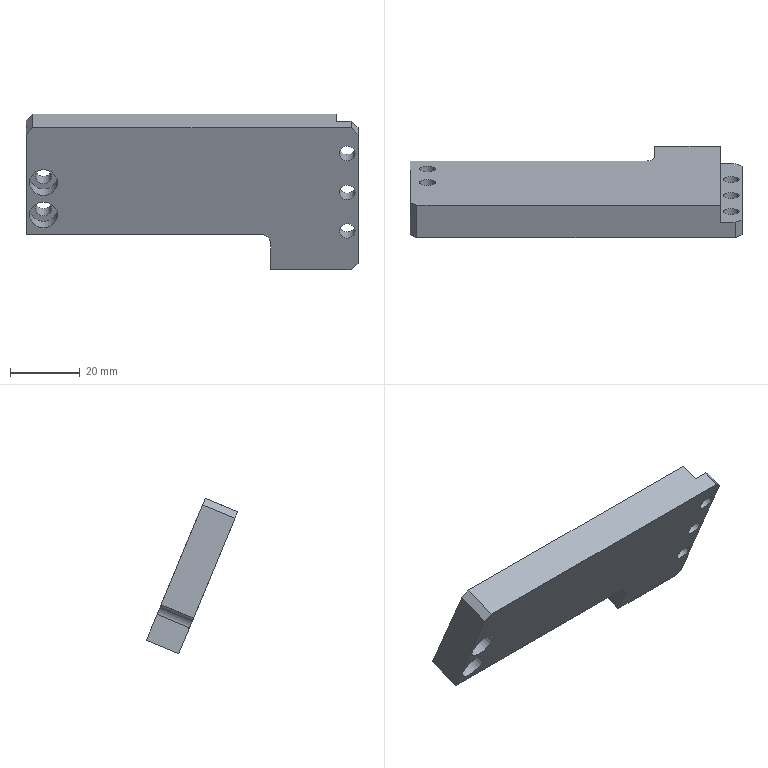Component | SolidWorks | 04-006BottomPlate-1 | 1 solid | 38 faces | box 95 x 26.13 x 44.47 mm | volume 31598 mm3 | cylinder 19 | plane 15 | cone 4 | commonest cylinder face diameters 4.5 x10 8 x4 3.3 x4 6 x1
build123d program:
from build123d import *

# Parameters (mm, degrees)
SKETCH1_W                                          = 95
SKETCH1_H                                          = 33
BOSS_EXTRUDE1_DEPTH                                = 10
M4_TAPPED_HOLE1_D                                  = 3.3
M4_TAPPED_HOLE1_DEPTH                              = 10.1
M4_TAPPED_HOLE1_TIP                                = 0.9914
HOLE_SIZE_ACCORDING_TO_TYPE_1_OF_HEX_S_D           = 4.5
HOLE_SIZE_ACCORDING_TO_TYPE_1_OF_HEX_S_DEPTH       = 10.1
HOLE_SIZE_ACCORDING_TO_TYPE_1_OF_HEX_S_CBORE_D     = 8
HOLE_SIZE_ACCORDING_TO_TYPE_1_OF_HEX_S_CBORE_DEPTH = 4.6
HOLE_SIZE_ACCORDING_TO_TYPE_1_OF_HEX_S_TIP         = 1.352
SKETCH11_W                                         = 25
SKETCH11_H                                         = 10
BOSS_EXTRUDE2_DEPTH                                = 11
SKETCH3_W                                          = 6.2
SKETCH3_H                                          = 44
CUT_EXTRUDE2_DEPTH                                 = 5.3
F_4_5_4_5_DIAMETER_HOLE1_D                         = 4.5
F_4_5_4_5_DIAMETER_HOLE1_DEPTH                     = 10.1
F_4_5_4_5_DIAMETER_HOLE1_TIP                       = 1.352
FILLET1_R                                          = 3
CHAMFER1_SIZE                                      = 2


with BuildPart() as part:
    # Sketch1 → Boss-Extrude1 (new body)
    with BuildSketch(Plane.XY):
        with Locations((47.5, 16.5)):
            Rectangle(SKETCH1_W, SKETCH1_H)
    extrude(amount=BOSS_EXTRUDE1_DEPTH)

    # M4 Tapped Hole1
    with Locations(Plane(origin=(0, 33, 0), x_dir=(1, 0, 0), z_dir=(0, 1, 0))):
        with Locations((60, -5), (80, -5)):
            Hole(M4_TAPPED_HOLE1_D / 2, depth=M4_TAPPED_HOLE1_DEPTH)
            with Locations((0, 0, -(M4_TAPPED_HOLE1_DEPTH + M4_TAPPED_HOLE1_TIP / 2))):  # 118° drill point
                Cone(0, M4_TAPPED_HOLE1_D / 2, M4_TAPPED_HOLE1_TIP, mode=Mode.SUBTRACT)

    # Hole Size _According to_ Type 1 of Hex S
    with Locations(Plane(origin=(0, 0, 10), x_dir=(-1, 0, 0), z_dir=(0, 0, 1))):
        with Locations((-90, -17), (-90, -27)):
            CounterBoreHole(HOLE_SIZE_ACCORDING_TO_TYPE_1_OF_HEX_S_D / 2, HOLE_SIZE_ACCORDING_TO_TYPE_1_OF_HEX_S_CBORE_D / 2, HOLE_SIZE_ACCORDING_TO_TYPE_1_OF_HEX_S_CBORE_DEPTH, depth=HOLE_SIZE_ACCORDING_TO_TYPE_1_OF_HEX_S_DEPTH)
            with Locations((0, 0, -(HOLE_SIZE_ACCORDING_TO_TYPE_1_OF_HEX_S_DEPTH + HOLE_SIZE_ACCORDING_TO_TYPE_1_OF_HEX_S_TIP / 2))):  # 118° drill point
                Cone(0, HOLE_SIZE_ACCORDING_TO_TYPE_1_OF_HEX_S_D / 2, HOLE_SIZE_ACCORDING_TO_TYPE_1_OF_HEX_S_TIP, mode=Mode.SUBTRACT)

    # Sketch11 → Boss-Extrude2 (add)
    with BuildSketch(Plane(origin=(0, 33, 0), x_dir=(1, 0, 0), z_dir=(0, 1, 0))):
        with Locations((12.5, -5)):
            Rectangle(SKETCH11_W, SKETCH11_H)
    extrude(amount=BOSS_EXTRUDE2_DEPTH)

    # Sketch3 → Cut-Extrude2 (cut)
    with BuildSketch(Plane(origin=(0, 0, 0), x_dir=(-1, 0, 0), z_dir=(0, 0, -1))):
        with Locations((-3.1, 22)):
            Rectangle(SKETCH3_W, SKETCH3_H)
    extrude(amount=-CUT_EXTRUDE2_DEPTH, mode=Mode.SUBTRACT)

    # 4.5 _4.5_ Diameter Hole1
    with Locations(Plane.XY.offset(10)):
        with Locations((3.1, 20), (3.1, 8), (3.1, 32)):
            Hole(F_4_5_4_5_DIAMETER_HOLE1_D / 2, depth=F_4_5_4_5_DIAMETER_HOLE1_DEPTH)
            with Locations((0, 0, -(F_4_5_4_5_DIAMETER_HOLE1_DEPTH + F_4_5_4_5_DIAMETER_HOLE1_TIP / 2))):  # 118° drill point
                Cone(0, F_4_5_4_5_DIAMETER_HOLE1_D / 2, F_4_5_4_5_DIAMETER_HOLE1_TIP, mode=Mode.SUBTRACT)

    # Fillet1
    fillet1_edges = [part.edges().sort_by_distance(p)[0] for p in [
        (25, 33, 5),
    ]]
    fillet(fillet1_edges, radius=FILLET1_R)

    # Chamfer1
    chamfer1_edges = [part.edges().sort_by_distance(p)[0] for p in [
        (0, 44, 7.65),
        (95, 0, 5),
        (0, 0, 7.65),
    ]]
    chamfer(chamfer1_edges, length=CHAMFER1_SIZE)


solid = part.part

# Placed as in the assembly
solid = solid.moved(Location((194.726, -33.174, 92.713), (112.584, 0, 180)))